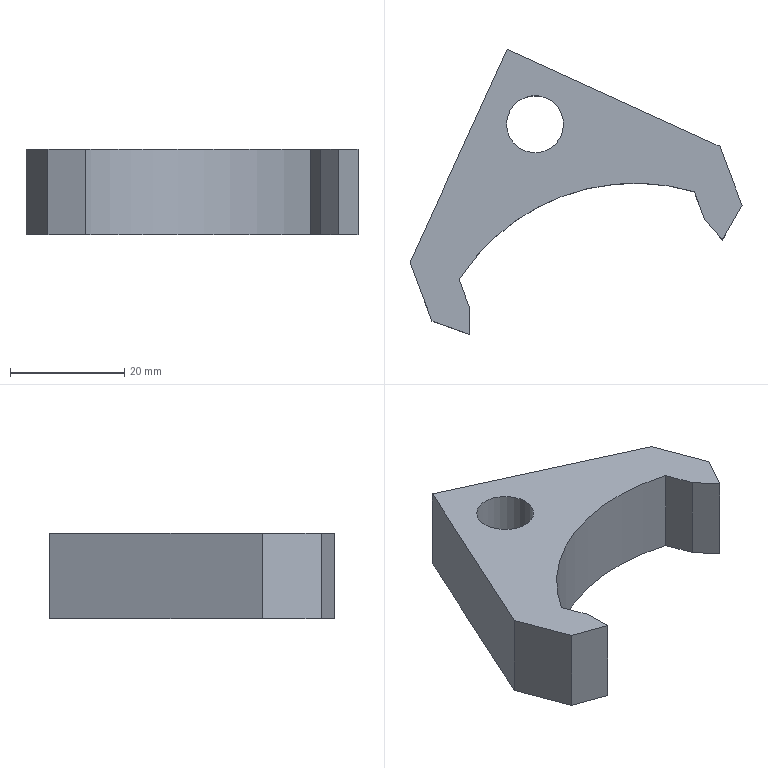Component | NX | PAWL | 1 solid | 14 faces | box 58.18 x 49.96 x 15 mm | volume 14780 mm3 | plane 12 | cylinder 2 | commonest cylinder face diameters 73 x1 10 x1
STEP:
#1=CARTESIAN_POINT('',(0.,0.,0.));
#2=DIRECTION('',(0.,0.,1.));
#3=DIRECTION('',(1.,0.,0.));
#4=AXIS2_PLACEMENT_3D('',#1,#2,#3);
#5=CARTESIAN_POINT('',(-19.22,66.93,312.973));
#6=VERTEX_POINT('',#5);
#7=CARTESIAN_POINT('',(18.099,49.923,312.973));
#8=VERTEX_POINT('',#7);
#9=CARTESIAN_POINT('',(-19.22,66.93,312.973));
#10=DIRECTION('',(0.91,-0.4147,0.));
#11=VECTOR('',#10,1.);
#12=LINE('',#9,#11);
#13=CARTESIAN_POINT('',(-19.22,66.93,327.973));
#14=DIRECTION('',(0.4147,0.91,0.));
#15=DIRECTION('',(-0.91,0.4147,0.));
#16=AXIS2_PLACEMENT_3D('',#13,#14,#15);
#17=PLANE('',#16);
#18=CARTESIAN_POINT('',(0.,-15.));
#19=DIRECTION('',(-1.,0.));
#20=VECTOR('',#19,1.);
#21=LINE('',#18,#20);
#22=(GEOMETRIC_REPRESENTATION_CONTEXT(2)PARAMETRIC_REPRESENTATION_CONTEXT()REPRESENTATION_CONTEXT('',''));
#23=DEFINITIONAL_REPRESENTATION('',(#21),#22);
#24=PCURVE('',#17,#23);
#25=CARTESIAN_POINT('',(3.193,6.983,312.973));
#26=DIRECTION('',(0.,0.,1.));
#27=DIRECTION('',(0.9367,0.3502,0.));
#28=AXIS2_PLACEMENT_3D('',#25,#26,#27);
#29=PLANE('',#28);
#30=CARTESIAN_POINT('',(0.,64.));
#31=DIRECTION('',(0.7071,-0.7071));
#32=VECTOR('',#31,1.);
#33=LINE('',#30,#32);
#34=(GEOMETRIC_REPRESENTATION_CONTEXT(2)PARAMETRIC_REPRESENTATION_CONTEXT()REPRESENTATION_CONTEXT('',''));
#35=DEFINITIONAL_REPRESENTATION('',(#33),#34);
#36=PCURVE('',#29,#35);
#37=SURFACE_CURVE('',#12,(#24,#36),.PCURVE_S1.);
#38=EDGE_CURVE('',#6,#8,#37,.T.);
#39=ORIENTED_EDGE('',*,*,#38,.F.);
#40=CARTESIAN_POINT('',(-19.22,66.93,327.973));
#41=VERTEX_POINT('',#40);
#42=CARTESIAN_POINT('',(-19.22,66.93,327.973));
#43=DIRECTION('',(0.,0.,-1.));
#44=VECTOR('',#43,1.);
#45=LINE('',#42,#44);
#46=CARTESIAN_POINT('',(0.,0.));
#47=DIRECTION('',(0.,-1.));
#48=VECTOR('',#47,1.);
#49=LINE('',#46,#48);
#50=(GEOMETRIC_REPRESENTATION_CONTEXT(2)PARAMETRIC_REPRESENTATION_CONTEXT()REPRESENTATION_CONTEXT('',''));
#51=DEFINITIONAL_REPRESENTATION('',(#49),#50);
#52=PCURVE('',#17,#51);
#53=CARTESIAN_POINT('',(-36.228,29.611,327.973));
#54=DIRECTION('',(-0.91,0.4147,0.));
#55=DIRECTION('',(-0.4147,-0.91,0.));
#56=AXIS2_PLACEMENT_3D('',#53,#54,#55);
#57=PLANE('',#56);
#58=CARTESIAN_POINT('',(-41.012,0.));
#59=DIRECTION('',(0.,-1.));
#60=VECTOR('',#59,1.);
#61=LINE('',#58,#60);
#62=(GEOMETRIC_REPRESENTATION_CONTEXT(2)PARAMETRIC_REPRESENTATION_CONTEXT()REPRESENTATION_CONTEXT('',''));
#63=DEFINITIONAL_REPRESENTATION('',(#61),#62);
#64=PCURVE('',#57,#63);
#65=SURFACE_CURVE('',#45,(#52,#64),.PCURVE_S1.);
#66=EDGE_CURVE('',#41,#6,#65,.T.);
#67=ORIENTED_EDGE('',*,*,#66,.F.);
#68=CARTESIAN_POINT('',(18.099,49.923,327.973));
#69=VERTEX_POINT('',#68);
#70=CARTESIAN_POINT('',(-19.22,66.93,327.973));
#71=DIRECTION('',(0.91,-0.4147,0.));
#72=VECTOR('',#71,1.);
#73=LINE('',#70,#72);
#74=CARTESIAN_POINT('',(0.,0.));
#75=DIRECTION('',(-1.,0.));
#76=VECTOR('',#75,1.);
#77=LINE('',#74,#76);
#78=(GEOMETRIC_REPRESENTATION_CONTEXT(2)PARAMETRIC_REPRESENTATION_CONTEXT()REPRESENTATION_CONTEXT('',''));
#79=DEFINITIONAL_REPRESENTATION('',(#77),#78);
#80=PCURVE('',#17,#79);
#81=CARTESIAN_POINT('',(3.193,6.983,327.973));
#82=DIRECTION('',(0.,0.,1.));
#83=DIRECTION('',(0.9367,0.3502,0.));
#84=AXIS2_PLACEMENT_3D('',#81,#82,#83);
#85=PLANE('',#84);
#86=CARTESIAN_POINT('',(0.,64.));
#87=DIRECTION('',(0.7071,-0.7071));
#88=VECTOR('',#87,1.);
#89=LINE('',#86,#88);
#90=(GEOMETRIC_REPRESENTATION_CONTEXT(2)PARAMETRIC_REPRESENTATION_CONTEXT()REPRESENTATION_CONTEXT('',''));
#91=DEFINITIONAL_REPRESENTATION('',(#89),#90);
#92=PCURVE('',#85,#91);
#93=SURFACE_CURVE('',#73,(#80,#92),.PCURVE_S1.);
#94=EDGE_CURVE('',#41,#69,#93,.T.);
#95=ORIENTED_EDGE('',*,*,#94,.T.);
#96=CARTESIAN_POINT('',(18.099,49.923,327.973));
#97=DIRECTION('',(0.,0.,-1.));
#98=VECTOR('',#97,1.);
#99=LINE('',#96,#98);
#100=CARTESIAN_POINT('',(-41.012,0.));
#101=DIRECTION('',(0.,-1.));
#102=VECTOR('',#101,1.);
#103=LINE('',#100,#102);
#104=(GEOMETRIC_REPRESENTATION_CONTEXT(2)PARAMETRIC_REPRESENTATION_CONTEXT()REPRESENTATION_CONTEXT('',''));
#105=DEFINITIONAL_REPRESENTATION('',(#103),#104);
#106=PCURVE('',#17,#105);
#107=CARTESIAN_POINT('',(18.099,49.923,327.973));
#108=DIRECTION('',(0.9367,0.3502,0.));
#109=DIRECTION('',(-0.3502,0.9367,0.));
#110=AXIS2_PLACEMENT_3D('',#107,#108,#109);
#111=PLANE('',#110);
#112=CARTESIAN_POINT('',(0.,0.));
#113=DIRECTION('',(0.,-1.));
#114=VECTOR('',#113,1.);
#115=LINE('',#112,#114);
#116=(GEOMETRIC_REPRESENTATION_CONTEXT(2)PARAMETRIC_REPRESENTATION_CONTEXT()REPRESENTATION_CONTEXT('',''));
#117=DEFINITIONAL_REPRESENTATION('',(#115),#116);
#118=PCURVE('',#111,#117);
#119=SURFACE_CURVE('',#99,(#106,#118),.PCURVE_S1.);
#120=EDGE_CURVE('',#69,#8,#119,.T.);
#121=ORIENTED_EDGE('',*,*,#120,.T.);
#122=EDGE_LOOP('',(#39,#67,#95,#121));
#123=FACE_BOUND('',#122,.T.);
#124=ADVANCED_FACE('',(#123),#17,.T.);
#125=CARTESIAN_POINT('',(21.952,39.619,312.973));
#126=VERTEX_POINT('',#125);
#127=CARTESIAN_POINT('',(18.099,49.923,312.973));
#128=DIRECTION('',(0.3502,-0.9367,0.));
#129=VECTOR('',#128,1.);
#130=LINE('',#127,#129);
#131=CARTESIAN_POINT('',(0.,-15.));
#132=DIRECTION('',(-1.,0.));
#133=VECTOR('',#132,1.);
#134=LINE('',#131,#133);
#135=(GEOMETRIC_REPRESENTATION_CONTEXT(2)PARAMETRIC_REPRESENTATION_CONTEXT()REPRESENTATION_CONTEXT('',''));
#136=DEFINITIONAL_REPRESENTATION('',(#134),#135);
#137=PCURVE('',#111,#136);
#138=CARTESIAN_POINT('',(29.,35.));
#139=DIRECTION('',(0.,-1.));
#140=VECTOR('',#139,1.);
#141=LINE('',#138,#140);
#142=(GEOMETRIC_REPRESENTATION_CONTEXT(2)PARAMETRIC_REPRESENTATION_CONTEXT()REPRESENTATION_CONTEXT('',''));
#143=DEFINITIONAL_REPRESENTATION('',(#141),#142);
#144=PCURVE('',#29,#143);
#145=SURFACE_CURVE('',#130,(#137,#144),.PCURVE_S1.);
#146=EDGE_CURVE('',#8,#126,#145,.T.);
#147=ORIENTED_EDGE('',*,*,#146,.F.);
#148=ORIENTED_EDGE('',*,*,#120,.F.);
#149=CARTESIAN_POINT('',(21.952,39.619,327.973));
#150=VERTEX_POINT('',#149);
#151=CARTESIAN_POINT('',(18.099,49.923,327.973));
#152=DIRECTION('',(0.3502,-0.9367,0.));
#153=VECTOR('',#152,1.);
#154=LINE('',#151,#153);
#155=CARTESIAN_POINT('',(0.,0.));
#156=DIRECTION('',(-1.,0.));
#157=VECTOR('',#156,1.);
#158=LINE('',#155,#157);
#159=(GEOMETRIC_REPRESENTATION_CONTEXT(2)PARAMETRIC_REPRESENTATION_CONTEXT()REPRESENTATION_CONTEXT('',''));
#160=DEFINITIONAL_REPRESENTATION('',(#158),#159);
#161=PCURVE('',#111,#160);
#162=CARTESIAN_POINT('',(29.,35.));
#163=DIRECTION('',(0.,-1.));
#164=VECTOR('',#163,1.);
#165=LINE('',#162,#164);
#166=(GEOMETRIC_REPRESENTATION_CONTEXT(2)PARAMETRIC_REPRESENTATION_CONTEXT()REPRESENTATION_CONTEXT('',''));
#167=DEFINITIONAL_REPRESENTATION('',(#165),#166);
#168=PCURVE('',#85,#167);
#169=SURFACE_CURVE('',#154,(#161,#168),.PCURVE_S1.);
#170=EDGE_CURVE('',#69,#150,#169,.T.);
#171=ORIENTED_EDGE('',*,*,#170,.T.);
#172=CARTESIAN_POINT('',(21.952,39.619,327.973));
#173=DIRECTION('',(0.,0.,-1.));
#174=VECTOR('',#173,1.);
#175=LINE('',#172,#174);
#176=CARTESIAN_POINT('',(-11.,0.));
#177=DIRECTION('',(0.,-1.));
#178=VECTOR('',#177,1.);
#179=LINE('',#176,#178);
#180=(GEOMETRIC_REPRESENTATION_CONTEXT(2)PARAMETRIC_REPRESENTATION_CONTEXT()REPRESENTATION_CONTEXT('',''));
#181=DEFINITIONAL_REPRESENTATION('',(#179),#180);
#182=PCURVE('',#111,#181);
#183=CARTESIAN_POINT('',(21.952,39.619,327.973));
#184=DIRECTION('',(0.8704,-0.4924,0.));
#185=DIRECTION('',(0.4924,0.8704,0.));
#186=AXIS2_PLACEMENT_3D('',#183,#184,#185);
#187=PLANE('',#186);
#188=CARTESIAN_POINT('',(0.,0.));
#189=DIRECTION('',(0.,-1.));
#190=VECTOR('',#189,1.);
#191=LINE('',#188,#190);
#192=(GEOMETRIC_REPRESENTATION_CONTEXT(2)PARAMETRIC_REPRESENTATION_CONTEXT()REPRESENTATION_CONTEXT('',''));
#193=DEFINITIONAL_REPRESENTATION('',(#191),#192);
#194=PCURVE('',#187,#193);
#195=SURFACE_CURVE('',#175,(#182,#194),.PCURVE_S1.);
#196=EDGE_CURVE('',#150,#126,#195,.T.);
#197=ORIENTED_EDGE('',*,*,#196,.T.);
#198=EDGE_LOOP('',(#147,#148,#171,#197));
#199=FACE_BOUND('',#198,.T.);
#200=ADVANCED_FACE('',(#199),#111,.T.);
#201=CARTESIAN_POINT('',(18.505,33.527,312.973));
#202=VERTEX_POINT('',#201);
#203=CARTESIAN_POINT('',(21.952,39.619,312.973));
#204=DIRECTION('',(-0.4924,-0.8704,0.));
#205=VECTOR('',#204,1.);
#206=LINE('',#203,#205);
#207=CARTESIAN_POINT('',(0.,-15.));
#208=DIRECTION('',(-1.,0.));
#209=VECTOR('',#208,1.);
#210=LINE('',#207,#209);
#211=(GEOMETRIC_REPRESENTATION_CONTEXT(2)PARAMETRIC_REPRESENTATION_CONTEXT()REPRESENTATION_CONTEXT('',''));
#212=DEFINITIONAL_REPRESENTATION('',(#210),#211);
#213=PCURVE('',#187,#212);
#214=CARTESIAN_POINT('',(29.,24.));
#215=DIRECTION('',(-0.766,-0.6428));
#216=VECTOR('',#215,1.);
#217=LINE('',#214,#216);
#218=(GEOMETRIC_REPRESENTATION_CONTEXT(2)PARAMETRIC_REPRESENTATION_CONTEXT()REPRESENTATION_CONTEXT('',''));
#219=DEFINITIONAL_REPRESENTATION('',(#217),#218);
#220=PCURVE('',#29,#219);
#221=SURFACE_CURVE('',#206,(#213,#220),.PCURVE_S1.);
#222=EDGE_CURVE('',#126,#202,#221,.T.);
#223=ORIENTED_EDGE('',*,*,#222,.F.);
#224=ORIENTED_EDGE('',*,*,#196,.F.);
#225=CARTESIAN_POINT('',(18.505,33.527,327.973));
#226=VERTEX_POINT('',#225);
#227=CARTESIAN_POINT('',(21.952,39.619,327.973));
#228=DIRECTION('',(-0.4924,-0.8704,0.));
#229=VECTOR('',#228,1.);
#230=LINE('',#227,#229);
#231=CARTESIAN_POINT('',(0.,0.));
#232=DIRECTION('',(-1.,0.));
#233=VECTOR('',#232,1.);
#234=LINE('',#231,#233);
#235=(GEOMETRIC_REPRESENTATION_CONTEXT(2)PARAMETRIC_REPRESENTATION_CONTEXT()REPRESENTATION_CONTEXT('',''));
#236=DEFINITIONAL_REPRESENTATION('',(#234),#235);
#237=PCURVE('',#187,#236);
#238=CARTESIAN_POINT('',(29.,24.));
#239=DIRECTION('',(-0.766,-0.6428));
#240=VECTOR('',#239,1.);
#241=LINE('',#238,#240);
#242=(GEOMETRIC_REPRESENTATION_CONTEXT(2)PARAMETRIC_REPRESENTATION_CONTEXT()REPRESENTATION_CONTEXT('',''));
#243=DEFINITIONAL_REPRESENTATION('',(#241),#242);
#244=PCURVE('',#85,#243);
#245=SURFACE_CURVE('',#230,(#237,#244),.PCURVE_S1.);
#246=EDGE_CURVE('',#150,#226,#245,.T.);
#247=ORIENTED_EDGE('',*,*,#246,.T.);
#248=CARTESIAN_POINT('',(18.505,33.527,327.973));
#249=DIRECTION('',(0.,0.,-1.));
#250=VECTOR('',#249,1.);
#251=LINE('',#248,#250);
#252=CARTESIAN_POINT('',(-7.,0.));
#253=DIRECTION('',(0.,-1.));
#254=VECTOR('',#253,1.);
#255=LINE('',#252,#254);
#256=(GEOMETRIC_REPRESENTATION_CONTEXT(2)PARAMETRIC_REPRESENTATION_CONTEXT()REPRESENTATION_CONTEXT('',''));
#257=DEFINITIONAL_REPRESENTATION('',(#255),#256);
#258=PCURVE('',#187,#257);
#259=CARTESIAN_POINT('',(18.505,33.527,327.973));
#260=DIRECTION('',(-0.7604,-0.6494,0.));
#261=DIRECTION('',(0.6494,-0.7604,0.));
#262=AXIS2_PLACEMENT_3D('',#259,#260,#261);
#263=PLANE('',#262);
#264=CARTESIAN_POINT('',(0.,0.));
#265=DIRECTION('',(0.,-1.));
#266=VECTOR('',#265,1.);
#267=LINE('',#264,#266);
#268=(GEOMETRIC_REPRESENTATION_CONTEXT(2)PARAMETRIC_REPRESENTATION_CONTEXT()REPRESENTATION_CONTEXT('',''));
#269=DEFINITIONAL_REPRESENTATION('',(#267),#268);
#270=PCURVE('',#263,#269);
#271=SURFACE_CURVE('',#251,(#258,#270),.PCURVE_S1.);
#272=EDGE_CURVE('',#226,#202,#271,.T.);
#273=ORIENTED_EDGE('',*,*,#272,.T.);
#274=EDGE_LOOP('',(#223,#224,#247,#273));
#275=FACE_BOUND('',#274,.T.);
#276=ADVANCED_FACE('',(#275),#187,.T.);
#277=CARTESIAN_POINT('',(15.395,37.168,312.973));
#278=VERTEX_POINT('',#277);
#279=CARTESIAN_POINT('',(18.505,33.527,312.973));
#280=DIRECTION('',(-0.6494,0.7604,0.));
#281=VECTOR('',#280,1.);
#282=LINE('',#279,#281);
#283=CARTESIAN_POINT('',(0.,-15.));
#284=DIRECTION('',(-1.,0.));
#285=VECTOR('',#284,1.);
#286=LINE('',#283,#285);
#287=(GEOMETRIC_REPRESENTATION_CONTEXT(2)PARAMETRIC_REPRESENTATION_CONTEXT()REPRESENTATION_CONTEXT('',''));
#288=DEFINITIONAL_REPRESENTATION('',(#286),#287);
#289=PCURVE('',#263,#288);
#290=CARTESIAN_POINT('',(23.638,19.5));
#291=DIRECTION('',(-0.342,0.9397));
#292=VECTOR('',#291,1.);
#293=LINE('',#290,#292);
#294=(GEOMETRIC_REPRESENTATION_CONTEXT(2)PARAMETRIC_REPRESENTATION_CONTEXT()REPRESENTATION_CONTEXT('',''));
#295=DEFINITIONAL_REPRESENTATION('',(#293),#294);
#296=PCURVE('',#29,#295);
#297=SURFACE_CURVE('',#282,(#289,#296),.PCURVE_S1.);
#298=EDGE_CURVE('',#202,#278,#297,.T.);
#299=ORIENTED_EDGE('',*,*,#298,.F.);
#300=ORIENTED_EDGE('',*,*,#272,.F.);
#301=CARTESIAN_POINT('',(15.395,37.168,327.973));
#302=VERTEX_POINT('',#301);
#303=CARTESIAN_POINT('',(18.505,33.527,327.973));
#304=DIRECTION('',(-0.6494,0.7604,0.));
#305=VECTOR('',#304,1.);
#306=LINE('',#303,#305);
#307=CARTESIAN_POINT('',(0.,0.));
#308=DIRECTION('',(-1.,0.));
#309=VECTOR('',#308,1.);
#310=LINE('',#307,#309);
#311=(GEOMETRIC_REPRESENTATION_CONTEXT(2)PARAMETRIC_REPRESENTATION_CONTEXT()REPRESENTATION_CONTEXT('',''));
#312=DEFINITIONAL_REPRESENTATION('',(#310),#311);
#313=PCURVE('',#263,#312);
#314=CARTESIAN_POINT('',(23.638,19.5));
#315=DIRECTION('',(-0.342,0.9397));
#316=VECTOR('',#315,1.);
#317=LINE('',#314,#316);
#318=(GEOMETRIC_REPRESENTATION_CONTEXT(2)PARAMETRIC_REPRESENTATION_CONTEXT()REPRESENTATION_CONTEXT('',''));
#319=DEFINITIONAL_REPRESENTATION('',(#317),#318);
#320=PCURVE('',#85,#319);
#321=SURFACE_CURVE('',#306,(#313,#320),.PCURVE_S1.);
#322=EDGE_CURVE('',#226,#302,#321,.T.);
#323=ORIENTED_EDGE('',*,*,#322,.T.);
#324=CARTESIAN_POINT('',(15.395,37.168,327.973));
#325=DIRECTION('',(0.,0.,-1.));
#326=VECTOR('',#325,1.);
#327=LINE('',#324,#326);
#328=CARTESIAN_POINT('',(-4.788,0.));
#329=DIRECTION('',(0.,-1.));
#330=VECTOR('',#329,1.);
#331=LINE('',#328,#330);
#332=(GEOMETRIC_REPRESENTATION_CONTEXT(2)PARAMETRIC_REPRESENTATION_CONTEXT()REPRESENTATION_CONTEXT('',''));
#333=DEFINITIONAL_REPRESENTATION('',(#331),#332);
#334=PCURVE('',#263,#333);
#335=CARTESIAN_POINT('',(15.395,37.168,327.973));
#336=DIRECTION('',(-0.9367,-0.3502,0.));
#337=DIRECTION('',(0.,0.,1.));
#338=AXIS2_PLACEMENT_3D('',#335,#336,#337);
#339=PLANE('',#338);
#340=CARTESIAN_POINT('',(0.,0.));
#341=DIRECTION('',(-1.,0.));
#342=VECTOR('',#341,1.);
#343=LINE('',#340,#342);
#344=(GEOMETRIC_REPRESENTATION_CONTEXT(2)PARAMETRIC_REPRESENTATION_CONTEXT()REPRESENTATION_CONTEXT('',''));
#345=DEFINITIONAL_REPRESENTATION('',(#343),#344);
#346=PCURVE('',#339,#345);
#347=SURFACE_CURVE('',#327,(#334,#346),.PCURVE_S1.);
#348=EDGE_CURVE('',#302,#278,#347,.T.);
#349=ORIENTED_EDGE('',*,*,#348,.T.);
#350=EDGE_LOOP('',(#299,#300,#323,#349));
#351=FACE_BOUND('',#350,.T.);
#352=ADVANCED_FACE('',(#351),#263,.T.);
#353=CARTESIAN_POINT('',(13.6,41.968,312.973));
#354=VERTEX_POINT('',#353);
#355=CARTESIAN_POINT('',(15.395,37.168,312.973));
#356=DIRECTION('',(-0.3502,0.9367,0.));
#357=VECTOR('',#356,1.);
#358=LINE('',#355,#357);
#359=CARTESIAN_POINT('',(-15.,0.));
#360=DIRECTION('',(0.,1.));
#361=VECTOR('',#360,1.);
#362=LINE('',#359,#361);
#363=(GEOMETRIC_REPRESENTATION_CONTEXT(2)PARAMETRIC_REPRESENTATION_CONTEXT()REPRESENTATION_CONTEXT('',''));
#364=DEFINITIONAL_REPRESENTATION('',(#362),#363);
#365=PCURVE('',#339,#364);
#366=CARTESIAN_POINT('',(22.,24.));
#367=DIRECTION('',(0.,1.));
#368=VECTOR('',#367,1.);
#369=LINE('',#366,#368);
#370=(GEOMETRIC_REPRESENTATION_CONTEXT(2)PARAMETRIC_REPRESENTATION_CONTEXT()REPRESENTATION_CONTEXT('',''));
#371=DEFINITIONAL_REPRESENTATION('',(#369),#370);
#372=PCURVE('',#29,#371);
#373=SURFACE_CURVE('',#358,(#365,#372),.PCURVE_S1.);
#374=EDGE_CURVE('',#278,#354,#373,.T.);
#375=ORIENTED_EDGE('',*,*,#374,.F.);
#376=ORIENTED_EDGE('',*,*,#348,.F.);
#377=CARTESIAN_POINT('',(13.6,41.968,327.973));
#378=VERTEX_POINT('',#377);
#379=CARTESIAN_POINT('',(15.395,37.168,327.973));
#380=DIRECTION('',(-0.3502,0.9367,0.));
#381=VECTOR('',#380,1.);
#382=LINE('',#379,#381);
#383=CARTESIAN_POINT('',(0.,0.));
#384=DIRECTION('',(0.,1.));
#385=VECTOR('',#384,1.);
#386=LINE('',#383,#385);
#387=(GEOMETRIC_REPRESENTATION_CONTEXT(2)PARAMETRIC_REPRESENTATION_CONTEXT()REPRESENTATION_CONTEXT('',''));
#388=DEFINITIONAL_REPRESENTATION('',(#386),#387);
#389=PCURVE('',#339,#388);
#390=CARTESIAN_POINT('',(22.,24.));
#391=DIRECTION('',(0.,1.));
#392=VECTOR('',#391,1.);
#393=LINE('',#390,#392);
#394=(GEOMETRIC_REPRESENTATION_CONTEXT(2)PARAMETRIC_REPRESENTATION_CONTEXT()REPRESENTATION_CONTEXT('',''));
#395=DEFINITIONAL_REPRESENTATION('',(#393),#394);
#396=PCURVE('',#85,#395);
#397=SURFACE_CURVE('',#382,(#389,#396),.PCURVE_S1.);
#398=EDGE_CURVE('',#302,#378,#397,.T.);
#399=ORIENTED_EDGE('',*,*,#398,.T.);
#400=CARTESIAN_POINT('',(13.6,41.968,327.973));
#401=DIRECTION('',(0.,0.,-1.));
#402=VECTOR('',#401,1.);
#403=LINE('',#400,#402);
#404=CARTESIAN_POINT('',(0.,5.125));
#405=DIRECTION('',(-1.,0.));
#406=VECTOR('',#405,1.);
#407=LINE('',#404,#406);
#408=(GEOMETRIC_REPRESENTATION_CONTEXT(2)PARAMETRIC_REPRESENTATION_CONTEXT()REPRESENTATION_CONTEXT('',''));
#409=DEFINITIONAL_REPRESENTATION('',(#407),#408);
#410=PCURVE('',#339,#409);
#411=CARTESIAN_POINT('',(3.193,6.983,327.973));
#412=DIRECTION('',(0.,0.,-1.));
#413=DIRECTION('',(-0.9367,-0.3502,0.));
#414=AXIS2_PLACEMENT_3D('',#411,#412,#413);
#415=CYLINDRICAL_SURFACE('',#414,36.5);
#416=CARTESIAN_POINT('',(2.218,0.));
#417=DIRECTION('',(0.,1.));
#418=VECTOR('',#417,1.);
#419=LINE('',#416,#418);
#420=(GEOMETRIC_REPRESENTATION_CONTEXT(2)PARAMETRIC_REPRESENTATION_CONTEXT()REPRESENTATION_CONTEXT('',''));
#421=DEFINITIONAL_REPRESENTATION('',(#419),#420);
#422=PCURVE('',#415,#421);
#423=SURFACE_CURVE('',#403,(#410,#422),.PCURVE_S1.);
#424=EDGE_CURVE('',#378,#354,#423,.T.);
#425=ORIENTED_EDGE('',*,*,#424,.T.);
#426=EDGE_LOOP('',(#375,#376,#399,#425));
#427=FACE_BOUND('',#426,.T.);
#428=ADVANCED_FACE('',(#427),#339,.T.);
#429=CARTESIAN_POINT('',(-27.613,26.559,327.973));
#430=VERTEX_POINT('',#429);
#431=CARTESIAN_POINT('',(-27.613,26.559,312.973));
#432=VERTEX_POINT('',#431);
#433=CARTESIAN_POINT('',(-27.613,26.559,327.973));
#434=DIRECTION('',(0.,0.,-1.));
#435=VECTOR('',#434,1.);
#436=LINE('',#433,#435);
#437=CARTESIAN_POINT('',(0.9239,0.));
#438=DIRECTION('',(0.,1.));
#439=VECTOR('',#438,1.);
#440=LINE('',#437,#439);
#441=(GEOMETRIC_REPRESENTATION_CONTEXT(2)PARAMETRIC_REPRESENTATION_CONTEXT()REPRESENTATION_CONTEXT('',''));
#442=DEFINITIONAL_REPRESENTATION('',(#440),#441);
#443=PCURVE('',#415,#442);
#444=CARTESIAN_POINT('',(-27.613,26.559,327.973));
#445=DIRECTION('',(0.9367,0.3502,0.));
#446=DIRECTION('',(0.,0.,-1.));
#447=AXIS2_PLACEMENT_3D('',#444,#445,#446);
#448=PLANE('',#447);
#449=CARTESIAN_POINT('',(0.,0.));
#450=DIRECTION('',(1.,0.));
#451=VECTOR('',#450,1.);
#452=LINE('',#449,#451);
#453=(GEOMETRIC_REPRESENTATION_CONTEXT(2)PARAMETRIC_REPRESENTATION_CONTEXT()REPRESENTATION_CONTEXT('',''));
#454=DEFINITIONAL_REPRESENTATION('',(#452),#453);
#455=PCURVE('',#448,#454);
#456=SURFACE_CURVE('',#436,(#443,#455),.PCURVE_S1.);
#457=EDGE_CURVE('',#430,#432,#456,.T.);
#458=ORIENTED_EDGE('',*,*,#457,.F.);
#459=CARTESIAN_POINT('',(3.193,6.983,327.973));
#460=DIRECTION('',(0.,0.,1.));
#461=DIRECTION('',(-0.3502,0.9367,0.));
#462=AXIS2_PLACEMENT_3D('',#459,#460,#461);
#463=CIRCLE('',#462,36.5);
#464=CARTESIAN_POINT('',(7.854,0.));
#465=DIRECTION('',(-1.,0.));
#466=VECTOR('',#465,1.);
#467=LINE('',#464,#466);
#468=(GEOMETRIC_REPRESENTATION_CONTEXT(2)PARAMETRIC_REPRESENTATION_CONTEXT()REPRESENTATION_CONTEXT('',''));
#469=DEFINITIONAL_REPRESENTATION('',(#467),#468);
#470=PCURVE('',#415,#469);
#471=CARTESIAN_POINT('',(0.,0.));
#472=DIRECTION('',(0.,1.));
#473=AXIS2_PLACEMENT_2D('',#471,#472);
#474=CIRCLE('',#473,36.5);
#475=(GEOMETRIC_REPRESENTATION_CONTEXT(2)PARAMETRIC_REPRESENTATION_CONTEXT()REPRESENTATION_CONTEXT('',''));
#476=DEFINITIONAL_REPRESENTATION('',(#474),#475);
#477=PCURVE('',#85,#476);
#478=SURFACE_CURVE('',#463,(#470,#477),.PCURVE_S1.);
#479=EDGE_CURVE('',#378,#430,#478,.T.);
#480=ORIENTED_EDGE('',*,*,#479,.F.);
#481=ORIENTED_EDGE('',*,*,#424,.T.);
#482=CARTESIAN_POINT('',(3.193,6.983,312.973));
#483=DIRECTION('',(0.,0.,1.));
#484=DIRECTION('',(-0.3502,0.9367,0.));
#485=AXIS2_PLACEMENT_3D('',#482,#483,#484);
#486=CIRCLE('',#485,36.5);
#487=CARTESIAN_POINT('',(7.854,15.));
#488=DIRECTION('',(-1.,0.));
#489=VECTOR('',#488,1.);
#490=LINE('',#487,#489);
#491=(GEOMETRIC_REPRESENTATION_CONTEXT(2)PARAMETRIC_REPRESENTATION_CONTEXT()REPRESENTATION_CONTEXT('',''));
#492=DEFINITIONAL_REPRESENTATION('',(#490),#491);
#493=PCURVE('',#415,#492);
#494=CARTESIAN_POINT('',(0.,0.));
#495=DIRECTION('',(0.,1.));
#496=AXIS2_PLACEMENT_2D('',#494,#495);
#497=CIRCLE('',#496,36.5);
#498=(GEOMETRIC_REPRESENTATION_CONTEXT(2)PARAMETRIC_REPRESENTATION_CONTEXT()REPRESENTATION_CONTEXT('',''));
#499=DEFINITIONAL_REPRESENTATION('',(#497),#498);
#500=PCURVE('',#29,#499);
#501=SURFACE_CURVE('',#486,(#493,#500),.PCURVE_S1.);
#502=EDGE_CURVE('',#354,#432,#501,.T.);
#503=ORIENTED_EDGE('',*,*,#502,.T.);
#504=EDGE_LOOP('',(#458,#480,#481,#503));
#505=FACE_BOUND('',#504,.F.);
#506=ADVANCED_FACE('',(#505),#415,.F.);
#507=CARTESIAN_POINT('',(-25.819,21.759,312.973));
#508=VERTEX_POINT('',#507);
#509=CARTESIAN_POINT('',(-27.613,26.559,312.973));
#510=DIRECTION('',(0.3502,-0.9367,0.));
#511=VECTOR('',#510,1.);
#512=LINE('',#509,#511);
#513=CARTESIAN_POINT('',(15.,0.));
#514=DIRECTION('',(0.,-1.));
#515=VECTOR('',#514,1.);
#516=LINE('',#513,#515);
#517=(GEOMETRIC_REPRESENTATION_CONTEXT(2)PARAMETRIC_REPRESENTATION_CONTEXT()REPRESENTATION_CONTEXT('',''));
#518=DEFINITIONAL_REPRESENTATION('',(#516),#517);
#519=PCURVE('',#448,#518);
#520=CARTESIAN_POINT('',(-22.,29.125));
#521=DIRECTION('',(0.,-1.));
#522=VECTOR('',#521,1.);
#523=LINE('',#520,#522);
#524=(GEOMETRIC_REPRESENTATION_CONTEXT(2)PARAMETRIC_REPRESENTATION_CONTEXT()REPRESENTATION_CONTEXT('',''));
#525=DEFINITIONAL_REPRESENTATION('',(#523),#524);
#526=PCURVE('',#29,#525);
#527=SURFACE_CURVE('',#512,(#519,#526),.PCURVE_S1.);
#528=EDGE_CURVE('',#432,#508,#527,.T.);
#529=ORIENTED_EDGE('',*,*,#528,.F.);
#530=ORIENTED_EDGE('',*,*,#457,.F.);
#531=CARTESIAN_POINT('',(-25.819,21.759,327.973));
#532=VERTEX_POINT('',#531);
#533=CARTESIAN_POINT('',(-27.613,26.559,327.973));
#534=DIRECTION('',(0.3502,-0.9367,0.));
#535=VECTOR('',#534,1.);
#536=LINE('',#533,#535);
#537=CARTESIAN_POINT('',(0.,0.));
#538=DIRECTION('',(0.,-1.));
#539=VECTOR('',#538,1.);
#540=LINE('',#537,#539);
#541=(GEOMETRIC_REPRESENTATION_CONTEXT(2)PARAMETRIC_REPRESENTATION_CONTEXT()REPRESENTATION_CONTEXT('',''));
#542=DEFINITIONAL_REPRESENTATION('',(#540),#541);
#543=PCURVE('',#448,#542);
#544=CARTESIAN_POINT('',(-22.,29.125));
#545=DIRECTION('',(0.,-1.));
#546=VECTOR('',#545,1.);
#547=LINE('',#544,#546);
#548=(GEOMETRIC_REPRESENTATION_CONTEXT(2)PARAMETRIC_REPRESENTATION_CONTEXT()REPRESENTATION_CONTEXT('',''));
#549=DEFINITIONAL_REPRESENTATION('',(#547),#548);
#550=PCURVE('',#85,#549);
#551=SURFACE_CURVE('',#536,(#543,#550),.PCURVE_S1.);
#552=EDGE_CURVE('',#430,#532,#551,.T.);
#553=ORIENTED_EDGE('',*,*,#552,.T.);
#554=CARTESIAN_POINT('',(-25.819,21.759,327.973));
#555=DIRECTION('',(0.,0.,-1.));
#556=VECTOR('',#555,1.);
#557=LINE('',#554,#556);
#558=CARTESIAN_POINT('',(0.,-5.125));
#559=DIRECTION('',(1.,0.));
#560=VECTOR('',#559,1.);
#561=LINE('',#558,#560);
#562=(GEOMETRIC_REPRESENTATION_CONTEXT(2)PARAMETRIC_REPRESENTATION_CONTEXT()REPRESENTATION_CONTEXT('',''));
#563=DEFINITIONAL_REPRESENTATION('',(#561),#562);
#564=PCURVE('',#448,#563);
#565=CARTESIAN_POINT('',(-25.819,21.759,327.973));
#566=DIRECTION('',(1.,0.008727,0.));
#567=DIRECTION('',(-0.008727,1.,0.));
#568=AXIS2_PLACEMENT_3D('',#565,#566,#567);
#569=PLANE('',#568);
#570=CARTESIAN_POINT('',(0.,0.));
#571=DIRECTION('',(0.,-1.));
#572=VECTOR('',#571,1.);
#573=LINE('',#570,#572);
#574=(GEOMETRIC_REPRESENTATION_CONTEXT(2)PARAMETRIC_REPRESENTATION_CONTEXT()REPRESENTATION_CONTEXT('',''));
#575=DEFINITIONAL_REPRESENTATION('',(#573),#574);
#576=PCURVE('',#569,#575);
#577=SURFACE_CURVE('',#557,(#564,#576),.PCURVE_S1.);
#578=EDGE_CURVE('',#532,#508,#577,.T.);
#579=ORIENTED_EDGE('',*,*,#578,.T.);
#580=EDGE_LOOP('',(#529,#530,#553,#579));
#581=FACE_BOUND('',#580,.T.);
#582=ADVANCED_FACE('',(#581),#448,.T.);
#583=CARTESIAN_POINT('',(-25.777,16.971,312.973));
#584=VERTEX_POINT('',#583);
#585=CARTESIAN_POINT('',(-25.819,21.759,312.973));
#586=DIRECTION('',(0.008727,-1.,0.));
#587=VECTOR('',#586,1.);
#588=LINE('',#585,#587);
#589=CARTESIAN_POINT('',(0.,-15.));
#590=DIRECTION('',(-1.,0.));
#591=VECTOR('',#590,1.);
#592=LINE('',#589,#591);
#593=(GEOMETRIC_REPRESENTATION_CONTEXT(2)PARAMETRIC_REPRESENTATION_CONTEXT()REPRESENTATION_CONTEXT('',''));
#594=DEFINITIONAL_REPRESENTATION('',(#592),#593);
#595=PCURVE('',#569,#594);
#596=CARTESIAN_POINT('',(-22.,24.));
#597=DIRECTION('',(-0.342,-0.9397));
#598=VECTOR('',#597,1.);
#599=LINE('',#596,#598);
#600=(GEOMETRIC_REPRESENTATION_CONTEXT(2)PARAMETRIC_REPRESENTATION_CONTEXT()REPRESENTATION_CONTEXT('',''));
#601=DEFINITIONAL_REPRESENTATION('',(#599),#600);
#602=PCURVE('',#29,#601);
#603=SURFACE_CURVE('',#588,(#595,#602),.PCURVE_S1.);
#604=EDGE_CURVE('',#508,#584,#603,.T.);
#605=ORIENTED_EDGE('',*,*,#604,.F.);
#606=ORIENTED_EDGE('',*,*,#578,.F.);
#607=CARTESIAN_POINT('',(-25.777,16.971,327.973));
#608=VERTEX_POINT('',#607);
#609=CARTESIAN_POINT('',(-25.819,21.759,327.973));
#610=DIRECTION('',(0.008727,-1.,0.));
#611=VECTOR('',#610,1.);
#612=LINE('',#609,#611);
#613=CARTESIAN_POINT('',(0.,0.));
#614=DIRECTION('',(-1.,0.));
#615=VECTOR('',#614,1.);
#616=LINE('',#613,#615);
#617=(GEOMETRIC_REPRESENTATION_CONTEXT(2)PARAMETRIC_REPRESENTATION_CONTEXT()REPRESENTATION_CONTEXT('',''));
#618=DEFINITIONAL_REPRESENTATION('',(#616),#617);
#619=PCURVE('',#569,#618);
#620=CARTESIAN_POINT('',(-22.,24.));
#621=DIRECTION('',(-0.342,-0.9397));
#622=VECTOR('',#621,1.);
#623=LINE('',#620,#622);
#624=(GEOMETRIC_REPRESENTATION_CONTEXT(2)PARAMETRIC_REPRESENTATION_CONTEXT()REPRESENTATION_CONTEXT('',''));
#625=DEFINITIONAL_REPRESENTATION('',(#623),#624);
#626=PCURVE('',#85,#625);
#627=SURFACE_CURVE('',#612,(#619,#626),.PCURVE_S1.);
#628=EDGE_CURVE('',#532,#608,#627,.T.);
#629=ORIENTED_EDGE('',*,*,#628,.T.);
#630=CARTESIAN_POINT('',(-25.777,16.971,327.973));
#631=DIRECTION('',(0.,0.,-1.));
#632=VECTOR('',#631,1.);
#633=LINE('',#630,#632);
#634=CARTESIAN_POINT('',(-4.788,0.));
#635=DIRECTION('',(0.,-1.));
#636=VECTOR('',#635,1.);
#637=LINE('',#634,#636);
#638=(GEOMETRIC_REPRESENTATION_CONTEXT(2)PARAMETRIC_REPRESENTATION_CONTEXT()REPRESENTATION_CONTEXT('',''));
#639=DEFINITIONAL_REPRESENTATION('',(#637),#638);
#640=PCURVE('',#569,#639);
#641=CARTESIAN_POINT('',(-25.777,16.971,327.973));
#642=DIRECTION('',(-0.3338,-0.9426,0.));
#643=DIRECTION('',(0.9426,-0.3338,0.));
#644=AXIS2_PLACEMENT_3D('',#641,#642,#643);
#645=PLANE('',#644);
#646=CARTESIAN_POINT('',(0.,0.));
#647=DIRECTION('',(0.,-1.));
#648=VECTOR('',#647,1.);
#649=LINE('',#646,#648);
#650=(GEOMETRIC_REPRESENTATION_CONTEXT(2)PARAMETRIC_REPRESENTATION_CONTEXT()REPRESENTATION_CONTEXT('',''));
#651=DEFINITIONAL_REPRESENTATION('',(#649),#650);
#652=PCURVE('',#645,#651);
#653=SURFACE_CURVE('',#633,(#640,#652),.PCURVE_S1.);
#654=EDGE_CURVE('',#608,#584,#653,.T.);
#655=ORIENTED_EDGE('',*,*,#654,.T.);
#656=EDGE_LOOP('',(#605,#606,#629,#655));
#657=FACE_BOUND('',#656,.T.);
#658=ADVANCED_FACE('',(#657),#569,.T.);
#659=CARTESIAN_POINT('',(-32.375,19.307,312.973));
#660=VERTEX_POINT('',#659);
#661=CARTESIAN_POINT('',(-25.777,16.971,312.973));
#662=DIRECTION('',(-0.9426,0.3338,0.));
#663=VECTOR('',#662,1.);
#664=LINE('',#661,#663);
#665=CARTESIAN_POINT('',(0.,-15.));
#666=DIRECTION('',(-1.,0.));
#667=VECTOR('',#666,1.);
#668=LINE('',#665,#667);
#669=(GEOMETRIC_REPRESENTATION_CONTEXT(2)PARAMETRIC_REPRESENTATION_CONTEXT()REPRESENTATION_CONTEXT('',''));
#670=DEFINITIONAL_REPRESENTATION('',(#668),#669);
#671=PCURVE('',#645,#670);
#672=CARTESIAN_POINT('',(-23.638,19.5));
#673=DIRECTION('',(-0.766,0.6428));
#674=VECTOR('',#673,1.);
#675=LINE('',#672,#674);
#676=(GEOMETRIC_REPRESENTATION_CONTEXT(2)PARAMETRIC_REPRESENTATION_CONTEXT()REPRESENTATION_CONTEXT('',''));
#677=DEFINITIONAL_REPRESENTATION('',(#675),#676);
#678=PCURVE('',#29,#677);
#679=SURFACE_CURVE('',#664,(#671,#678),.PCURVE_S1.);
#680=EDGE_CURVE('',#584,#660,#679,.T.);
#681=ORIENTED_EDGE('',*,*,#680,.F.);
#682=ORIENTED_EDGE('',*,*,#654,.F.);
#683=CARTESIAN_POINT('',(-32.375,19.307,327.973));
#684=VERTEX_POINT('',#683);
#685=CARTESIAN_POINT('',(-25.777,16.971,327.973));
#686=DIRECTION('',(-0.9426,0.3338,0.));
#687=VECTOR('',#686,1.);
#688=LINE('',#685,#687);
#689=CARTESIAN_POINT('',(0.,0.));
#690=DIRECTION('',(-1.,0.));
#691=VECTOR('',#690,1.);
#692=LINE('',#689,#691);
#693=(GEOMETRIC_REPRESENTATION_CONTEXT(2)PARAMETRIC_REPRESENTATION_CONTEXT()REPRESENTATION_CONTEXT('',''));
#694=DEFINITIONAL_REPRESENTATION('',(#692),#693);
#695=PCURVE('',#645,#694);
#696=CARTESIAN_POINT('',(-23.638,19.5));
#697=DIRECTION('',(-0.766,0.6428));
#698=VECTOR('',#697,1.);
#699=LINE('',#696,#698);
#700=(GEOMETRIC_REPRESENTATION_CONTEXT(2)PARAMETRIC_REPRESENTATION_CONTEXT()REPRESENTATION_CONTEXT('',''));
#701=DEFINITIONAL_REPRESENTATION('',(#699),#700);
#702=PCURVE('',#85,#701);
#703=SURFACE_CURVE('',#688,(#695,#702),.PCURVE_S1.);
#704=EDGE_CURVE('',#608,#684,#703,.T.);
#705=ORIENTED_EDGE('',*,*,#704,.T.);
#706=CARTESIAN_POINT('',(-32.375,19.307,327.973));
#707=DIRECTION('',(0.,0.,-1.));
#708=VECTOR('',#707,1.);
#709=LINE('',#706,#708);
#710=CARTESIAN_POINT('',(-7.,0.));
#711=DIRECTION('',(0.,-1.));
#712=VECTOR('',#711,1.);
#713=LINE('',#710,#712);
#714=(GEOMETRIC_REPRESENTATION_CONTEXT(2)PARAMETRIC_REPRESENTATION_CONTEXT()REPRESENTATION_CONTEXT('',''));
#715=DEFINITIONAL_REPRESENTATION('',(#713),#714);
#716=PCURVE('',#645,#715);
#717=CARTESIAN_POINT('',(-32.375,19.307,327.973));
#718=DIRECTION('',(-0.9367,-0.3502,0.));
#719=DIRECTION('',(0.3502,-0.9367,0.));
#720=AXIS2_PLACEMENT_3D('',#717,#718,#719);
#721=PLANE('',#720);
#722=CARTESIAN_POINT('',(0.,0.));
#723=DIRECTION('',(0.,-1.));
#724=VECTOR('',#723,1.);
#725=LINE('',#722,#724);
#726=(GEOMETRIC_REPRESENTATION_CONTEXT(2)PARAMETRIC_REPRESENTATION_CONTEXT()REPRESENTATION_CONTEXT('',''));
#727=DEFINITIONAL_REPRESENTATION('',(#725),#726);
#728=PCURVE('',#721,#727);
#729=SURFACE_CURVE('',#709,(#716,#728),.PCURVE_S1.);
#730=EDGE_CURVE('',#684,#660,#729,.T.);
#731=ORIENTED_EDGE('',*,*,#730,.T.);
#732=EDGE_LOOP('',(#681,#682,#705,#731));
#733=FACE_BOUND('',#732,.T.);
#734=ADVANCED_FACE('',(#733),#645,.T.);
#735=CARTESIAN_POINT('',(-36.228,29.611,312.973));
#736=VERTEX_POINT('',#735);
#737=CARTESIAN_POINT('',(-32.375,19.307,312.973));
#738=DIRECTION('',(-0.3502,0.9367,0.));
#739=VECTOR('',#738,1.);
#740=LINE('',#737,#739);
#741=CARTESIAN_POINT('',(0.,-15.));
#742=DIRECTION('',(-1.,0.));
#743=VECTOR('',#742,1.);
#744=LINE('',#741,#743);
#745=(GEOMETRIC_REPRESENTATION_CONTEXT(2)PARAMETRIC_REPRESENTATION_CONTEXT()REPRESENTATION_CONTEXT('',''));
#746=DEFINITIONAL_REPRESENTATION('',(#744),#745);
#747=PCURVE('',#721,#746);
#748=CARTESIAN_POINT('',(-29.,24.));
#749=DIRECTION('',(-0.,1.));
#750=VECTOR('',#749,1.);
#751=LINE('',#748,#750);
#752=(GEOMETRIC_REPRESENTATION_CONTEXT(2)PARAMETRIC_REPRESENTATION_CONTEXT()REPRESENTATION_CONTEXT('',''));
#753=DEFINITIONAL_REPRESENTATION('',(#751),#752);
#754=PCURVE('',#29,#753);
#755=SURFACE_CURVE('',#740,(#747,#754),.PCURVE_S1.);
#756=EDGE_CURVE('',#660,#736,#755,.T.);
#757=ORIENTED_EDGE('',*,*,#756,.F.);
#758=ORIENTED_EDGE('',*,*,#730,.F.);
#759=CARTESIAN_POINT('',(-36.228,29.611,327.973));
#760=VERTEX_POINT('',#759);
#761=CARTESIAN_POINT('',(-32.375,19.307,327.973));
#762=DIRECTION('',(-0.3502,0.9367,0.));
#763=VECTOR('',#762,1.);
#764=LINE('',#761,#763);
#765=CARTESIAN_POINT('',(0.,0.));
#766=DIRECTION('',(-1.,0.));
#767=VECTOR('',#766,1.);
#768=LINE('',#765,#767);
#769=(GEOMETRIC_REPRESENTATION_CONTEXT(2)PARAMETRIC_REPRESENTATION_CONTEXT()REPRESENTATION_CONTEXT('',''));
#770=DEFINITIONAL_REPRESENTATION('',(#768),#769);
#771=PCURVE('',#721,#770);
#772=CARTESIAN_POINT('',(-29.,24.));
#773=DIRECTION('',(-0.,1.));
#774=VECTOR('',#773,1.);
#775=LINE('',#772,#774);
#776=(GEOMETRIC_REPRESENTATION_CONTEXT(2)PARAMETRIC_REPRESENTATION_CONTEXT()REPRESENTATION_CONTEXT('',''));
#777=DEFINITIONAL_REPRESENTATION('',(#775),#776);
#778=PCURVE('',#85,#777);
#779=SURFACE_CURVE('',#764,(#771,#778),.PCURVE_S1.);
#780=EDGE_CURVE('',#684,#760,#779,.T.);
#781=ORIENTED_EDGE('',*,*,#780,.T.);
#782=CARTESIAN_POINT('',(-36.228,29.611,327.973));
#783=DIRECTION('',(0.,0.,-1.));
#784=VECTOR('',#783,1.);
#785=LINE('',#782,#784);
#786=CARTESIAN_POINT('',(-11.,0.));
#787=DIRECTION('',(0.,-1.));
#788=VECTOR('',#787,1.);
#789=LINE('',#786,#788);
#790=(GEOMETRIC_REPRESENTATION_CONTEXT(2)PARAMETRIC_REPRESENTATION_CONTEXT()REPRESENTATION_CONTEXT('',''));
#791=DEFINITIONAL_REPRESENTATION('',(#789),#790);
#792=PCURVE('',#721,#791);
#793=CARTESIAN_POINT('',(0.,0.));
#794=DIRECTION('',(0.,-1.));
#795=VECTOR('',#794,1.);
#796=LINE('',#793,#795);
#797=(GEOMETRIC_REPRESENTATION_CONTEXT(2)PARAMETRIC_REPRESENTATION_CONTEXT()REPRESENTATION_CONTEXT('',''));
#798=DEFINITIONAL_REPRESENTATION('',(#796),#797);
#799=PCURVE('',#57,#798);
#800=SURFACE_CURVE('',#785,(#792,#799),.PCURVE_S1.);
#801=EDGE_CURVE('',#760,#736,#800,.T.);
#802=ORIENTED_EDGE('',*,*,#801,.T.);
#803=EDGE_LOOP('',(#757,#758,#781,#802));
#804=FACE_BOUND('',#803,.T.);
#805=ADVANCED_FACE('',(#804),#721,.T.);
#806=CARTESIAN_POINT('',(-36.228,29.611,312.973));
#807=DIRECTION('',(0.4147,0.91,0.));
#808=VECTOR('',#807,1.);
#809=LINE('',#806,#808);
#810=CARTESIAN_POINT('',(0.,-15.));
#811=DIRECTION('',(-1.,0.));
#812=VECTOR('',#811,1.);
#813=LINE('',#810,#812);
#814=(GEOMETRIC_REPRESENTATION_CONTEXT(2)PARAMETRIC_REPRESENTATION_CONTEXT()REPRESENTATION_CONTEXT('',''));
#815=DEFINITIONAL_REPRESENTATION('',(#813),#814);
#816=PCURVE('',#57,#815);
#817=CARTESIAN_POINT('',(-29.,35.));
#818=DIRECTION('',(0.7071,0.7071));
#819=VECTOR('',#818,1.);
#820=LINE('',#817,#819);
#821=(GEOMETRIC_REPRESENTATION_CONTEXT(2)PARAMETRIC_REPRESENTATION_CONTEXT()REPRESENTATION_CONTEXT('',''));
#822=DEFINITIONAL_REPRESENTATION('',(#820),#821);
#823=PCURVE('',#29,#822);
#824=SURFACE_CURVE('',#809,(#816,#823),.PCURVE_S1.);
#825=EDGE_CURVE('',#736,#6,#824,.T.);
#826=ORIENTED_EDGE('',*,*,#825,.F.);
#827=ORIENTED_EDGE('',*,*,#801,.F.);
#828=CARTESIAN_POINT('',(-36.228,29.611,327.973));
#829=DIRECTION('',(0.4147,0.91,0.));
#830=VECTOR('',#829,1.);
#831=LINE('',#828,#830);
#832=CARTESIAN_POINT('',(0.,0.));
#833=DIRECTION('',(-1.,0.));
#834=VECTOR('',#833,1.);
#835=LINE('',#832,#834);
#836=(GEOMETRIC_REPRESENTATION_CONTEXT(2)PARAMETRIC_REPRESENTATION_CONTEXT()REPRESENTATION_CONTEXT('',''));
#837=DEFINITIONAL_REPRESENTATION('',(#835),#836);
#838=PCURVE('',#57,#837);
#839=CARTESIAN_POINT('',(-29.,35.));
#840=DIRECTION('',(0.7071,0.7071));
#841=VECTOR('',#840,1.);
#842=LINE('',#839,#841);
#843=(GEOMETRIC_REPRESENTATION_CONTEXT(2)PARAMETRIC_REPRESENTATION_CONTEXT()REPRESENTATION_CONTEXT('',''));
#844=DEFINITIONAL_REPRESENTATION('',(#842),#843);
#845=PCURVE('',#85,#844);
#846=SURFACE_CURVE('',#831,(#838,#845),.PCURVE_S1.);
#847=EDGE_CURVE('',#760,#41,#846,.T.);
#848=ORIENTED_EDGE('',*,*,#847,.T.);
#849=ORIENTED_EDGE('',*,*,#66,.T.);
#850=EDGE_LOOP('',(#826,#827,#848,#849));
#851=FACE_BOUND('',#850,.T.);
#852=ADVANCED_FACE('',(#851),#57,.T.);
#853=CARTESIAN_POINT('',(-16.068,58.5,327.973));
#854=VERTEX_POINT('',#853);
#855=CARTESIAN_POINT('',(-14.317,53.817,327.973));
#856=DIRECTION('',(0.,0.,1.));
#857=DIRECTION('',(-0.3502,0.9367,0.));
#858=AXIS2_PLACEMENT_3D('',#855,#856,#857);
#859=CIRCLE('',#858,5.);
#860=CARTESIAN_POINT('',(-14.317,53.817,327.973));
#861=DIRECTION('',(0.,0.,-1.));
#862=DIRECTION('',(-0.9367,-0.3502,0.));
#863=AXIS2_PLACEMENT_3D('',#860,#861,#862);
#864=CYLINDRICAL_SURFACE('',#863,5.);
#865=CARTESIAN_POINT('',(7.854,0.));
#866=DIRECTION('',(-1.,0.));
#867=VECTOR('',#866,1.);
#868=LINE('',#865,#867);
#869=(GEOMETRIC_REPRESENTATION_CONTEXT(2)PARAMETRIC_REPRESENTATION_CONTEXT()REPRESENTATION_CONTEXT('',''));
#870=DEFINITIONAL_REPRESENTATION('',(#868),#869);
#871=PCURVE('',#864,#870);
#872=CARTESIAN_POINT('',(-0.,50.));
#873=DIRECTION('',(0.,1.));
#874=AXIS2_PLACEMENT_2D('',#872,#873);
#875=CIRCLE('',#874,5.);
#876=(GEOMETRIC_REPRESENTATION_CONTEXT(2)PARAMETRIC_REPRESENTATION_CONTEXT()REPRESENTATION_CONTEXT('',''));
#877=DEFINITIONAL_REPRESENTATION('',(#875),#876);
#878=PCURVE('',#85,#877);
#879=SURFACE_CURVE('',#859,(#871,#878),.PCURVE_S1.);
#880=EDGE_CURVE('',#854,#854,#879,.T.);
#881=ORIENTED_EDGE('',*,*,#880,.F.);
#882=CARTESIAN_POINT('',(-16.068,58.5,312.973));
#883=VERTEX_POINT('',#882);
#884=CARTESIAN_POINT('',(-16.068,58.5,327.973));
#885=CARTESIAN_POINT('',(-16.068,58.5,312.973));
#886=B_SPLINE_CURVE_WITH_KNOTS('',1,(#884,#885),.UNSPECIFIED.,.F.,.F.,(2,2),(0.,15.),.PIECEWISE_BEZIER_KNOTS.);
#887=CARTESIAN_POINT('',(7.854,0.));
#888=DIRECTION('',(0.,1.));
#889=VECTOR('',#888,1.);
#890=LINE('',#887,#889);
#891=(GEOMETRIC_REPRESENTATION_CONTEXT(2)PARAMETRIC_REPRESENTATION_CONTEXT()REPRESENTATION_CONTEXT('',''));
#892=DEFINITIONAL_REPRESENTATION('',(#890),#891);
#893=PCURVE('',#864,#892);
#894=CARTESIAN_POINT('',(1.571,0.));
#895=DIRECTION('',(0.,1.));
#896=VECTOR('',#895,1.);
#897=LINE('',#894,#896);
#898=(GEOMETRIC_REPRESENTATION_CONTEXT(2)PARAMETRIC_REPRESENTATION_CONTEXT()REPRESENTATION_CONTEXT('',''));
#899=DEFINITIONAL_REPRESENTATION('',(#897),#898);
#900=PCURVE('',#864,#899);
#901=SEAM_CURVE('',#886,(#893,#900),.PCURVE_S1.);
#902=EDGE_CURVE('',#854,#883,#901,.T.);
#903=ORIENTED_EDGE('',*,*,#902,.T.);
#904=CARTESIAN_POINT('',(-14.317,53.817,312.973));
#905=DIRECTION('',(0.,0.,1.));
#906=DIRECTION('',(-0.3502,0.9367,0.));
#907=AXIS2_PLACEMENT_3D('',#904,#905,#906);
#908=CIRCLE('',#907,5.);
#909=CARTESIAN_POINT('',(7.854,15.));
#910=DIRECTION('',(-1.,0.));
#911=VECTOR('',#910,1.);
#912=LINE('',#909,#911);
#913=(GEOMETRIC_REPRESENTATION_CONTEXT(2)PARAMETRIC_REPRESENTATION_CONTEXT()REPRESENTATION_CONTEXT('',''));
#914=DEFINITIONAL_REPRESENTATION('',(#912),#913);
#915=PCURVE('',#864,#914);
#916=CARTESIAN_POINT('',(-0.,50.));
#917=DIRECTION('',(0.,1.));
#918=AXIS2_PLACEMENT_2D('',#916,#917);
#919=CIRCLE('',#918,5.);
#920=(GEOMETRIC_REPRESENTATION_CONTEXT(2)PARAMETRIC_REPRESENTATION_CONTEXT()REPRESENTATION_CONTEXT('',''));
#921=DEFINITIONAL_REPRESENTATION('',(#919),#920);
#922=PCURVE('',#29,#921);
#923=SURFACE_CURVE('',#908,(#915,#922),.PCURVE_S1.);
#924=EDGE_CURVE('',#883,#883,#923,.T.);
#925=ORIENTED_EDGE('',*,*,#924,.T.);
#926=ORIENTED_EDGE('',*,*,#902,.F.);
#927=EDGE_LOOP('',(#881,#903,#925,#926));
#928=FACE_BOUND('',#927,.F.);
#929=ADVANCED_FACE('',(#928),#864,.F.);
#930=ORIENTED_EDGE('',*,*,#94,.F.);
#931=ORIENTED_EDGE('',*,*,#847,.F.);
#932=ORIENTED_EDGE('',*,*,#780,.F.);
#933=ORIENTED_EDGE('',*,*,#704,.F.);
#934=ORIENTED_EDGE('',*,*,#628,.F.);
#935=ORIENTED_EDGE('',*,*,#552,.F.);
#936=ORIENTED_EDGE('',*,*,#479,.F.);
#937=ORIENTED_EDGE('',*,*,#398,.F.);
#938=ORIENTED_EDGE('',*,*,#322,.F.);
#939=ORIENTED_EDGE('',*,*,#246,.F.);
#940=ORIENTED_EDGE('',*,*,#170,.F.);
#941=EDGE_LOOP('',(#930,#931,#932,#933,#934,#935,#936,#937,#938,#939,#940));
#942=FACE_BOUND('',#941,.T.);
#943=ORIENTED_EDGE('',*,*,#880,.F.);
#944=EDGE_LOOP('',(#943));
#945=FACE_BOUND('',#944,.T.);
#946=ADVANCED_FACE('',(#942,#945),#85,.T.);
#947=ORIENTED_EDGE('',*,*,#38,.T.);
#948=ORIENTED_EDGE('',*,*,#146,.T.);
#949=ORIENTED_EDGE('',*,*,#222,.T.);
#950=ORIENTED_EDGE('',*,*,#298,.T.);
#951=ORIENTED_EDGE('',*,*,#374,.T.);
#952=ORIENTED_EDGE('',*,*,#502,.T.);
#953=ORIENTED_EDGE('',*,*,#528,.T.);
#954=ORIENTED_EDGE('',*,*,#604,.T.);
#955=ORIENTED_EDGE('',*,*,#680,.T.);
#956=ORIENTED_EDGE('',*,*,#756,.T.);
#957=ORIENTED_EDGE('',*,*,#825,.T.);
#958=EDGE_LOOP('',(#947,#948,#949,#950,#951,#952,#953,#954,#955,#956,#957));
#959=FACE_BOUND('',#958,.T.);
#960=ORIENTED_EDGE('',*,*,#924,.T.);
#961=EDGE_LOOP('',(#960));
#962=FACE_BOUND('',#961,.T.);
#963=ADVANCED_FACE('',(#959,#962),#29,.F.);
#964=CLOSED_SHELL('',(#124,#200,#276,#352,#428,#506,#582,#658,#734,#805,#852,#929,#946,#963));
#965=MANIFOLD_SOLID_BREP('',#964);
#966=(LENGTH_UNIT()NAMED_UNIT(*)SI_UNIT(.MILLI.,.METRE.));
#967=UNCERTAINTY_MEASURE_WITH_UNIT(LENGTH_MEASURE(0.000001),#966,'','');
#968=(NAMED_UNIT(*)PLANE_ANGLE_UNIT()SI_UNIT($,.RADIAN.));
#969=(NAMED_UNIT(*)SI_UNIT($,.STERADIAN.)SOLID_ANGLE_UNIT());
#970=(GEOMETRIC_REPRESENTATION_CONTEXT(3)GLOBAL_UNCERTAINTY_ASSIGNED_CONTEXT((#967))GLOBAL_UNIT_ASSIGNED_CONTEXT((#966,#968,#969))REPRESENTATION_CONTEXT('',''));
#971=ADVANCED_BREP_SHAPE_REPRESENTATION('',(#4,#965),#970);